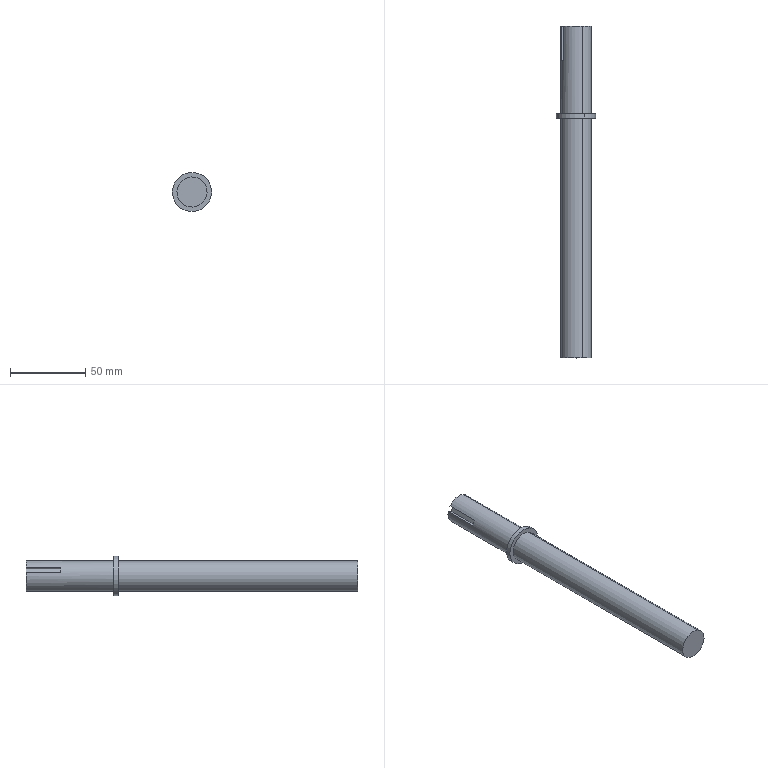Component | SolidWorks | LX-TSJ-07-1 | 1 solid | 18 faces | box 26 x 220 x 26 mm | volume 69227 mm3 | plane 12 | cylinder 6 | commonest cylinder face diameters 20 x4 26 x2
STEP:
#1=COLOUR_RGB('',0.7922,0.8196,0.9333);
#2=FILL_AREA_STYLE_COLOUR('',#1);
#3=FILL_AREA_STYLE('',(#2));
#4=SURFACE_STYLE_FILL_AREA(#3);
#5=SURFACE_SIDE_STYLE('',(#4));
#6=SURFACE_STYLE_USAGE(.BOTH.,#5);
#7=PRESENTATION_STYLE_ASSIGNMENT((#6));
#8=CARTESIAN_POINT('',(-12.95,-27.531,-15.901));
#9=VERTEX_POINT('',#8);
#10=CARTESIAN_POINT('',(-13.272,-27.531,-16.62));
#11=VERTEX_POINT('',#10);
#12=CARTESIAN_POINT('',(-13.111,-27.531,-16.26));
#13=DIRECTION('',(-0.,1.,0.));
#14=DIRECTION('',(0.4092,0.,0.9125));
#15=AXIS2_PLACEMENT_3D('',#12,#13,#14);
#16=CIRCLE('',#15,0.3937);
#17=EDGE_CURVE('',#9,#11,#16,.T.);
#18=ORIENTED_EDGE('',*,*,#17,.T.);
#19=CARTESIAN_POINT('',(-13.272,-21.272,-16.62));
#20=VERTEX_POINT('',#19);
#21=CARTESIAN_POINT('',(-13.272,-18.87,-16.62));
#22=DIRECTION('',(-0.,1.,0.));
#23=VECTOR('',#22,39.37);
#24=LINE('',#21,#23);
#25=EDGE_CURVE('',#11,#20,#24,.T.);
#26=ORIENTED_EDGE('',*,*,#25,.T.);
#27=CARTESIAN_POINT('',(-12.95,-21.272,-15.901));
#28=VERTEX_POINT('',#27);
#29=CARTESIAN_POINT('',(-13.111,-21.272,-16.26));
#30=DIRECTION('',(0.,-1.,-0.));
#31=DIRECTION('',(0.4092,0.,0.9125));
#32=AXIS2_PLACEMENT_3D('',#29,#30,#31);
#33=CIRCLE('',#32,0.3937);
#34=EDGE_CURVE('',#20,#28,#33,.T.);
#35=ORIENTED_EDGE('',*,*,#34,.T.);
#36=CARTESIAN_POINT('',(-12.95,-18.87,-15.901));
#37=DIRECTION('',(-0.,1.,0.));
#38=VECTOR('',#37,39.37);
#39=LINE('',#36,#38);
#40=EDGE_CURVE('',#9,#28,#39,.T.);
#41=ORIENTED_EDGE('',*,*,#40,.F.);
#42=EDGE_LOOP('',(#18,#26,#35,#41));
#43=FACE_OUTER_BOUND('',#42,.T.);
#44=CARTESIAN_POINT('',(-13.111,-18.87,-16.26));
#45=DIRECTION('',(-0.,1.,0.));
#46=DIRECTION('',(0.4092,-0.,0.9125));
#47=AXIS2_PLACEMENT_3D('',#44,#45,#46);
#48=CYLINDRICAL_SURFACE('',#47,0.3937);
#49=ADVANCED_FACE('',(#43),#48,.T.);
#50=CARTESIAN_POINT('',(-13.32,-21.272,-16.727));
#51=VERTEX_POINT('',#50);
#52=CARTESIAN_POINT('',(-12.902,-21.272,-15.793));
#53=VERTEX_POINT('',#52);
#54=CARTESIAN_POINT('',(-13.111,-21.272,-16.26));
#55=DIRECTION('',(0.,-1.,-0.));
#56=DIRECTION('',(0.4092,0.,0.9125));
#57=AXIS2_PLACEMENT_3D('',#54,#55,#56);
#58=CIRCLE('',#57,0.5118);
#59=EDGE_CURVE('',#51,#53,#58,.T.);
#60=ORIENTED_EDGE('',*,*,#59,.F.);
#61=CARTESIAN_POINT('',(-13.32,-21.154,-16.727));
#62=VERTEX_POINT('',#61);
#63=CARTESIAN_POINT('',(-13.32,-18.87,-16.727));
#64=DIRECTION('',(-0.,1.,0.));
#65=VECTOR('',#64,39.37);
#66=LINE('',#63,#65);
#67=EDGE_CURVE('',#51,#62,#66,.T.);
#68=ORIENTED_EDGE('',*,*,#67,.T.);
#69=CARTESIAN_POINT('',(-12.902,-21.154,-15.793));
#70=VERTEX_POINT('',#69);
#71=CARTESIAN_POINT('',(-13.111,-21.154,-16.26));
#72=DIRECTION('',(0.,-1.,-0.));
#73=DIRECTION('',(0.4092,0.,0.9125));
#74=AXIS2_PLACEMENT_3D('',#71,#72,#73);
#75=CIRCLE('',#74,0.5118);
#76=EDGE_CURVE('',#62,#70,#75,.T.);
#77=ORIENTED_EDGE('',*,*,#76,.T.);
#78=CARTESIAN_POINT('',(-12.902,-18.87,-15.793));
#79=DIRECTION('',(-0.,1.,0.));
#80=VECTOR('',#79,39.37);
#81=LINE('',#78,#80);
#82=EDGE_CURVE('',#53,#70,#81,.T.);
#83=ORIENTED_EDGE('',*,*,#82,.F.);
#84=EDGE_LOOP('',(#60,#68,#77,#83));
#85=FACE_OUTER_BOUND('',#84,.T.);
#86=CARTESIAN_POINT('',(-13.111,-18.87,-16.26));
#87=DIRECTION('',(-0.,1.,0.));
#88=DIRECTION('',(0.4092,-0.,0.9125));
#89=AXIS2_PLACEMENT_3D('',#86,#87,#88);
#90=CYLINDRICAL_SURFACE('',#89,0.5118);
#91=ADVANCED_FACE('',(#85),#90,.T.);
#92=CARTESIAN_POINT('',(-13.272,-21.154,-16.62));
#93=VERTEX_POINT('',#92);
#94=CARTESIAN_POINT('',(-12.95,-21.154,-15.901));
#95=VERTEX_POINT('',#94);
#96=CARTESIAN_POINT('',(-13.111,-21.154,-16.26));
#97=DIRECTION('',(0.,-1.,-0.));
#98=DIRECTION('',(0.4092,0.,0.9125));
#99=AXIS2_PLACEMENT_3D('',#96,#97,#98);
#100=CIRCLE('',#99,0.3937);
#101=EDGE_CURVE('',#93,#95,#100,.T.);
#102=ORIENTED_EDGE('',*,*,#101,.F.);
#103=CARTESIAN_POINT('',(-13.272,-18.87,-16.62));
#104=VERTEX_POINT('',#103);
#105=CARTESIAN_POINT('',(-13.272,-18.87,-16.62));
#106=DIRECTION('',(-0.,1.,0.));
#107=VECTOR('',#106,39.37);
#108=LINE('',#105,#107);
#109=EDGE_CURVE('',#93,#104,#108,.T.);
#110=ORIENTED_EDGE('',*,*,#109,.T.);
#111=CARTESIAN_POINT('',(-12.791,-18.87,-16.49));
#112=VERTEX_POINT('',#111);
#113=CARTESIAN_POINT('',(-13.111,-18.87,-16.26));
#114=DIRECTION('',(0.,-1.,-0.));
#115=DIRECTION('',(0.4092,-0.,0.9125));
#116=AXIS2_PLACEMENT_3D('',#113,#114,#115);
#117=CIRCLE('',#116,0.3937);
#118=EDGE_CURVE('',#104,#112,#117,.T.);
#119=ORIENTED_EDGE('',*,*,#118,.T.);
#120=CARTESIAN_POINT('',(-12.791,-19.774,-16.49));
#121=VERTEX_POINT('',#120);
#122=CARTESIAN_POINT('',(-12.791,-18.87,-16.49));
#123=DIRECTION('',(0.,-1.,-0.));
#124=VECTOR('',#123,39.37);
#125=LINE('',#122,#124);
#126=EDGE_CURVE('',#112,#121,#125,.T.);
#127=ORIENTED_EDGE('',*,*,#126,.T.);
#128=CARTESIAN_POINT('',(-12.727,-19.774,-16.346));
#129=VERTEX_POINT('',#128);
#130=CARTESIAN_POINT('',(-13.111,-19.774,-16.26));
#131=DIRECTION('',(0.,-1.,-0.));
#132=DIRECTION('',(0.4092,0.,0.9125));
#133=AXIS2_PLACEMENT_3D('',#130,#131,#132);
#134=CIRCLE('',#133,0.3937);
#135=EDGE_CURVE('',#121,#129,#134,.T.);
#136=ORIENTED_EDGE('',*,*,#135,.T.);
#137=CARTESIAN_POINT('',(-12.727,-18.87,-16.346));
#138=VERTEX_POINT('',#137);
#139=CARTESIAN_POINT('',(-12.727,-18.87,-16.346));
#140=DIRECTION('',(-0.,1.,0.));
#141=VECTOR('',#140,39.37);
#142=LINE('',#139,#141);
#143=EDGE_CURVE('',#129,#138,#142,.T.);
#144=ORIENTED_EDGE('',*,*,#143,.T.);
#145=CARTESIAN_POINT('',(-12.95,-18.87,-15.901));
#146=VERTEX_POINT('',#145);
#147=CARTESIAN_POINT('',(-13.111,-18.87,-16.26));
#148=DIRECTION('',(0.,-1.,-0.));
#149=DIRECTION('',(0.4092,-0.,0.9125));
#150=AXIS2_PLACEMENT_3D('',#147,#148,#149);
#151=CIRCLE('',#150,0.3937);
#152=EDGE_CURVE('',#138,#146,#151,.T.);
#153=ORIENTED_EDGE('',*,*,#152,.T.);
#154=CARTESIAN_POINT('',(-12.95,-18.87,-15.901));
#155=DIRECTION('',(-0.,1.,0.));
#156=VECTOR('',#155,39.37);
#157=LINE('',#154,#156);
#158=EDGE_CURVE('',#95,#146,#157,.T.);
#159=ORIENTED_EDGE('',*,*,#158,.F.);
#160=EDGE_LOOP('',(#102,#110,#119,#127,#136,#144,#153,#159));
#161=FACE_OUTER_BOUND('',#160,.T.);
#162=CARTESIAN_POINT('',(-13.111,-18.87,-16.26));
#163=DIRECTION('',(-0.,1.,0.));
#164=DIRECTION('',(0.4092,-0.,0.9125));
#165=AXIS2_PLACEMENT_3D('',#162,#163,#164);
#166=CYLINDRICAL_SURFACE('',#165,0.3937);
#167=ADVANCED_FACE('',(#161),#166,.T.);
#168=ORIENTED_EDGE('',*,*,#25,.F.);
#169=CARTESIAN_POINT('',(-13.111,-27.531,-16.26));
#170=DIRECTION('',(-0.,1.,0.));
#171=DIRECTION('',(0.4092,0.,0.9125));
#172=AXIS2_PLACEMENT_3D('',#169,#170,#171);
#173=CIRCLE('',#172,0.3937);
#174=EDGE_CURVE('',#11,#9,#173,.T.);
#175=ORIENTED_EDGE('',*,*,#174,.T.);
#176=ORIENTED_EDGE('',*,*,#40,.T.);
#177=CARTESIAN_POINT('',(-13.111,-21.272,-16.26));
#178=DIRECTION('',(0.,-1.,-0.));
#179=DIRECTION('',(0.4092,0.,0.9125));
#180=AXIS2_PLACEMENT_3D('',#177,#178,#179);
#181=CIRCLE('',#180,0.3937);
#182=EDGE_CURVE('',#28,#20,#181,.T.);
#183=ORIENTED_EDGE('',*,*,#182,.T.);
#184=EDGE_LOOP('',(#168,#175,#176,#183));
#185=FACE_OUTER_BOUND('',#184,.T.);
#186=CARTESIAN_POINT('',(-13.111,-18.87,-16.26));
#187=DIRECTION('',(-0.,1.,0.));
#188=DIRECTION('',(0.4092,-0.,0.9125));
#189=AXIS2_PLACEMENT_3D('',#186,#187,#188);
#190=CYLINDRICAL_SURFACE('',#189,0.3937);
#191=ADVANCED_FACE('',(#185),#190,.T.);
#192=CARTESIAN_POINT('',(-13.111,-21.272,-16.26));
#193=DIRECTION('',(0.,-1.,-0.));
#194=DIRECTION('',(0.4092,0.,0.9125));
#195=AXIS2_PLACEMENT_3D('',#192,#193,#194);
#196=CIRCLE('',#195,0.5118);
#197=EDGE_CURVE('',#53,#51,#196,.T.);
#198=ORIENTED_EDGE('',*,*,#197,.T.);
#199=ORIENTED_EDGE('',*,*,#59,.T.);
#200=EDGE_LOOP('',(#198,#199));
#201=FACE_OUTER_BOUND('',#200,.T.);
#202=ORIENTED_EDGE('',*,*,#182,.F.);
#203=ORIENTED_EDGE('',*,*,#34,.F.);
#204=EDGE_LOOP('',(#202,#203));
#205=FACE_BOUND('',#204,.T.);
#206=CARTESIAN_POINT('',(-13.954,-21.272,-15.882));
#207=DIRECTION('',(0.,-1.,-0.));
#208=DIRECTION('',(-0.4092,0.,-0.9125));
#209=AXIS2_PLACEMENT_3D('',#206,#207,#208);
#210=PLANE('',#209);
#211=ADVANCED_FACE('',(#201,#205),#210,.T.);
#212=ORIENTED_EDGE('',*,*,#17,.F.);
#213=ORIENTED_EDGE('',*,*,#174,.F.);
#214=EDGE_LOOP('',(#212,#213));
#215=FACE_OUTER_BOUND('',#214,.T.);
#216=CARTESIAN_POINT('',(-13.954,-27.531,-15.882));
#217=DIRECTION('',(0.,-1.,-0.));
#218=DIRECTION('',(-0.4092,0.,-0.9125));
#219=AXIS2_PLACEMENT_3D('',#216,#217,#218);
#220=PLANE('',#219);
#221=ADVANCED_FACE('',(#215),#220,.T.);
#222=ORIENTED_EDGE('',*,*,#67,.F.);
#223=ORIENTED_EDGE('',*,*,#197,.F.);
#224=ORIENTED_EDGE('',*,*,#82,.T.);
#225=CARTESIAN_POINT('',(-13.111,-21.154,-16.26));
#226=DIRECTION('',(0.,-1.,-0.));
#227=DIRECTION('',(0.4092,0.,0.9125));
#228=AXIS2_PLACEMENT_3D('',#225,#226,#227);
#229=CIRCLE('',#228,0.5118);
#230=EDGE_CURVE('',#70,#62,#229,.T.);
#231=ORIENTED_EDGE('',*,*,#230,.T.);
#232=EDGE_LOOP('',(#222,#223,#224,#231));
#233=FACE_OUTER_BOUND('',#232,.T.);
#234=CARTESIAN_POINT('',(-13.111,-18.87,-16.26));
#235=DIRECTION('',(-0.,1.,0.));
#236=DIRECTION('',(0.4092,-0.,0.9125));
#237=AXIS2_PLACEMENT_3D('',#234,#235,#236);
#238=CYLINDRICAL_SURFACE('',#237,0.5118);
#239=ADVANCED_FACE('',(#233),#238,.T.);
#240=CARTESIAN_POINT('',(-13.111,-21.154,-16.26));
#241=DIRECTION('',(0.,-1.,-0.));
#242=DIRECTION('',(0.4092,0.,0.9125));
#243=AXIS2_PLACEMENT_3D('',#240,#241,#242);
#244=CIRCLE('',#243,0.3937);
#245=EDGE_CURVE('',#95,#93,#244,.T.);
#246=ORIENTED_EDGE('',*,*,#245,.T.);
#247=ORIENTED_EDGE('',*,*,#101,.T.);
#248=EDGE_LOOP('',(#246,#247));
#249=FACE_BOUND('',#248,.T.);
#250=ORIENTED_EDGE('',*,*,#230,.F.);
#251=ORIENTED_EDGE('',*,*,#76,.F.);
#252=EDGE_LOOP('',(#250,#251));
#253=FACE_OUTER_BOUND('',#252,.T.);
#254=CARTESIAN_POINT('',(-13.954,-21.154,-15.882));
#255=DIRECTION('',(-0.,1.,0.));
#256=DIRECTION('',(0.4092,-0.,0.9125));
#257=AXIS2_PLACEMENT_3D('',#254,#255,#256);
#258=PLANE('',#257);
#259=ADVANCED_FACE('',(#249,#253),#258,.T.);
#260=ORIENTED_EDGE('',*,*,#109,.F.);
#261=ORIENTED_EDGE('',*,*,#245,.F.);
#262=ORIENTED_EDGE('',*,*,#158,.T.);
#263=CARTESIAN_POINT('',(-13.431,-18.87,-16.031));
#264=VERTEX_POINT('',#263);
#265=CARTESIAN_POINT('',(-13.111,-18.87,-16.26));
#266=DIRECTION('',(0.,-1.,-0.));
#267=DIRECTION('',(0.4092,-0.,0.9125));
#268=AXIS2_PLACEMENT_3D('',#265,#266,#267);
#269=CIRCLE('',#268,0.3937);
#270=EDGE_CURVE('',#146,#264,#269,.T.);
#271=ORIENTED_EDGE('',*,*,#270,.T.);
#272=CARTESIAN_POINT('',(-13.431,-19.774,-16.031));
#273=VERTEX_POINT('',#272);
#274=CARTESIAN_POINT('',(-13.431,-18.87,-16.031));
#275=DIRECTION('',(0.,-1.,-0.));
#276=VECTOR('',#275,39.37);
#277=LINE('',#274,#276);
#278=EDGE_CURVE('',#264,#273,#277,.T.);
#279=ORIENTED_EDGE('',*,*,#278,.T.);
#280=CARTESIAN_POINT('',(-13.495,-19.774,-16.174));
#281=VERTEX_POINT('',#280);
#282=CARTESIAN_POINT('',(-13.111,-19.774,-16.26));
#283=DIRECTION('',(0.,-1.,-0.));
#284=DIRECTION('',(0.4092,0.,0.9125));
#285=AXIS2_PLACEMENT_3D('',#282,#283,#284);
#286=CIRCLE('',#285,0.3937);
#287=EDGE_CURVE('',#273,#281,#286,.T.);
#288=ORIENTED_EDGE('',*,*,#287,.T.);
#289=CARTESIAN_POINT('',(-13.495,-18.87,-16.174));
#290=VERTEX_POINT('',#289);
#291=CARTESIAN_POINT('',(-13.495,-18.87,-16.174));
#292=DIRECTION('',(-0.,1.,0.));
#293=VECTOR('',#292,39.37);
#294=LINE('',#291,#293);
#295=EDGE_CURVE('',#281,#290,#294,.T.);
#296=ORIENTED_EDGE('',*,*,#295,.T.);
#297=CARTESIAN_POINT('',(-13.111,-18.87,-16.26));
#298=DIRECTION('',(0.,-1.,-0.));
#299=DIRECTION('',(0.4092,-0.,0.9125));
#300=AXIS2_PLACEMENT_3D('',#297,#298,#299);
#301=CIRCLE('',#300,0.3937);
#302=EDGE_CURVE('',#290,#104,#301,.T.);
#303=ORIENTED_EDGE('',*,*,#302,.T.);
#304=EDGE_LOOP('',(#260,#261,#262,#271,#279,#288,#296,#303));
#305=FACE_OUTER_BOUND('',#304,.T.);
#306=CARTESIAN_POINT('',(-13.111,-18.87,-16.26));
#307=DIRECTION('',(-0.,1.,0.));
#308=DIRECTION('',(0.4092,-0.,0.9125));
#309=AXIS2_PLACEMENT_3D('',#306,#307,#308);
#310=CYLINDRICAL_SURFACE('',#309,0.3937);
#311=ADVANCED_FACE('',(#305),#310,.T.);
#312=CARTESIAN_POINT('',(-12.827,-18.87,-16.301));
#313=VERTEX_POINT('',#312);
#314=CARTESIAN_POINT('',(-12.892,-18.87,-16.445));
#315=VERTEX_POINT('',#314);
#316=CARTESIAN_POINT('',(-12.859,-18.87,-16.373));
#317=DIRECTION('',(-0.4092,0.,-0.9125));
#318=VECTOR('',#317,39.37);
#319=LINE('',#316,#318);
#320=EDGE_CURVE('',#313,#315,#319,.T.);
#321=ORIENTED_EDGE('',*,*,#320,.T.);
#322=CARTESIAN_POINT('',(-13.986,-18.87,-15.954));
#323=DIRECTION('',(0.9125,0.,-0.4092));
#324=VECTOR('',#323,39.37);
#325=LINE('',#322,#324);
#326=EDGE_CURVE('',#315,#112,#325,.T.);
#327=ORIENTED_EDGE('',*,*,#326,.T.);
#328=ORIENTED_EDGE('',*,*,#118,.F.);
#329=ORIENTED_EDGE('',*,*,#302,.F.);
#330=CARTESIAN_POINT('',(-13.395,-18.87,-16.22));
#331=VERTEX_POINT('',#330);
#332=CARTESIAN_POINT('',(-13.986,-18.87,-15.954));
#333=DIRECTION('',(0.9125,0.,-0.4092));
#334=VECTOR('',#333,39.37);
#335=LINE('',#332,#334);
#336=EDGE_CURVE('',#290,#331,#335,.T.);
#337=ORIENTED_EDGE('',*,*,#336,.T.);
#338=CARTESIAN_POINT('',(-13.33,-18.87,-16.076));
#339=VERTEX_POINT('',#338);
#340=CARTESIAN_POINT('',(-13.362,-18.87,-16.148));
#341=DIRECTION('',(0.4092,-0.,0.9125));
#342=VECTOR('',#341,39.37);
#343=LINE('',#340,#342);
#344=EDGE_CURVE('',#331,#339,#343,.T.);
#345=ORIENTED_EDGE('',*,*,#344,.T.);
#346=CARTESIAN_POINT('',(-13.922,-18.87,-15.81));
#347=DIRECTION('',(-0.9125,-0.,0.4092));
#348=VECTOR('',#347,39.37);
#349=LINE('',#346,#348);
#350=EDGE_CURVE('',#339,#264,#349,.T.);
#351=ORIENTED_EDGE('',*,*,#350,.T.);
#352=ORIENTED_EDGE('',*,*,#270,.F.);
#353=ORIENTED_EDGE('',*,*,#152,.F.);
#354=CARTESIAN_POINT('',(-13.922,-18.87,-15.81));
#355=DIRECTION('',(-0.9125,-0.,0.4092));
#356=VECTOR('',#355,39.37);
#357=LINE('',#354,#356);
#358=EDGE_CURVE('',#138,#313,#357,.T.);
#359=ORIENTED_EDGE('',*,*,#358,.T.);
#360=EDGE_LOOP('',(#321,#327,#328,#329,#337,#345,#351,#352,#353,#359));
#361=FACE_OUTER_BOUND('',#360,.T.);
#362=CARTESIAN_POINT('',(-13.954,-18.87,-15.882));
#363=DIRECTION('',(-0.,1.,0.));
#364=DIRECTION('',(0.4092,-0.,0.9125));
#365=AXIS2_PLACEMENT_3D('',#362,#363,#364);
#366=PLANE('',#365);
#367=ADVANCED_FACE('',(#361),#366,.T.);
#368=CARTESIAN_POINT('',(-13.395,-19.774,-16.22));
#369=VERTEX_POINT('',#368);
#370=CARTESIAN_POINT('',(-13.986,-19.774,-15.954));
#371=DIRECTION('',(0.9125,0.,-0.4092));
#372=VECTOR('',#371,39.37);
#373=LINE('',#370,#372);
#374=EDGE_CURVE('',#281,#369,#373,.T.);
#375=ORIENTED_EDGE('',*,*,#374,.T.);
#376=CARTESIAN_POINT('',(-13.395,-19.774,-16.22));
#377=DIRECTION('',(-0.,1.,0.));
#378=VECTOR('',#377,39.37);
#379=LINE('',#376,#378);
#380=EDGE_CURVE('',#369,#331,#379,.T.);
#381=ORIENTED_EDGE('',*,*,#380,.T.);
#382=ORIENTED_EDGE('',*,*,#336,.F.);
#383=ORIENTED_EDGE('',*,*,#295,.F.);
#384=EDGE_LOOP('',(#375,#381,#382,#383));
#385=FACE_OUTER_BOUND('',#384,.T.);
#386=CARTESIAN_POINT('',(-13.986,-19.774,-15.954));
#387=DIRECTION('',(0.4092,-0.,0.9125));
#388=DIRECTION('',(0.,-1.,-0.));
#389=AXIS2_PLACEMENT_3D('',#386,#387,#388);
#390=PLANE('',#389);
#391=ADVANCED_FACE('',(#385),#390,.T.);
#392=CARTESIAN_POINT('',(-13.33,-19.774,-16.076));
#393=VERTEX_POINT('',#392);
#394=CARTESIAN_POINT('',(-13.362,-19.774,-16.148));
#395=DIRECTION('',(-0.4092,0.,-0.9125));
#396=VECTOR('',#395,39.37);
#397=LINE('',#394,#396);
#398=EDGE_CURVE('',#393,#369,#397,.T.);
#399=ORIENTED_EDGE('',*,*,#398,.T.);
#400=ORIENTED_EDGE('',*,*,#374,.F.);
#401=ORIENTED_EDGE('',*,*,#287,.F.);
#402=CARTESIAN_POINT('',(-13.922,-19.774,-15.81));
#403=DIRECTION('',(0.9125,0.,-0.4092));
#404=VECTOR('',#403,39.37);
#405=LINE('',#402,#404);
#406=EDGE_CURVE('',#273,#393,#405,.T.);
#407=ORIENTED_EDGE('',*,*,#406,.T.);
#408=EDGE_LOOP('',(#399,#400,#401,#407));
#409=FACE_OUTER_BOUND('',#408,.T.);
#410=CARTESIAN_POINT('',(-13.954,-19.774,-15.882));
#411=DIRECTION('',(-0.,1.,0.));
#412=DIRECTION('',(0.4092,-0.,0.9125));
#413=AXIS2_PLACEMENT_3D('',#410,#411,#412);
#414=PLANE('',#413);
#415=ADVANCED_FACE('',(#409),#414,.T.);
#416=CARTESIAN_POINT('',(-13.33,-19.774,-16.076));
#417=DIRECTION('',(-0.,1.,0.));
#418=VECTOR('',#417,39.37);
#419=LINE('',#416,#418);
#420=EDGE_CURVE('',#393,#339,#419,.T.);
#421=ORIENTED_EDGE('',*,*,#420,.F.);
#422=ORIENTED_EDGE('',*,*,#406,.F.);
#423=ORIENTED_EDGE('',*,*,#278,.F.);
#424=ORIENTED_EDGE('',*,*,#350,.F.);
#425=EDGE_LOOP('',(#421,#422,#423,#424));
#426=FACE_OUTER_BOUND('',#425,.T.);
#427=CARTESIAN_POINT('',(-13.922,-19.774,-15.81));
#428=DIRECTION('',(0.4092,-0.,0.9125));
#429=DIRECTION('',(0.,-1.,-0.));
#430=AXIS2_PLACEMENT_3D('',#427,#428,#429);
#431=PLANE('',#430);
#432=ADVANCED_FACE('',(#426),#431,.F.);
#433=ORIENTED_EDGE('',*,*,#143,.F.);
#434=CARTESIAN_POINT('',(-12.827,-19.774,-16.301));
#435=VERTEX_POINT('',#434);
#436=CARTESIAN_POINT('',(-13.922,-19.774,-15.81));
#437=DIRECTION('',(0.9125,0.,-0.4092));
#438=VECTOR('',#437,39.37);
#439=LINE('',#436,#438);
#440=EDGE_CURVE('',#435,#129,#439,.T.);
#441=ORIENTED_EDGE('',*,*,#440,.F.);
#442=CARTESIAN_POINT('',(-12.827,-19.774,-16.301));
#443=DIRECTION('',(0.,-1.,-0.));
#444=VECTOR('',#443,39.37);
#445=LINE('',#442,#444);
#446=EDGE_CURVE('',#313,#435,#445,.T.);
#447=ORIENTED_EDGE('',*,*,#446,.F.);
#448=ORIENTED_EDGE('',*,*,#358,.F.);
#449=EDGE_LOOP('',(#433,#441,#447,#448));
#450=FACE_OUTER_BOUND('',#449,.T.);
#451=CARTESIAN_POINT('',(-13.922,-19.774,-15.81));
#452=DIRECTION('',(0.4092,-0.,0.9125));
#453=DIRECTION('',(0.,-1.,-0.));
#454=AXIS2_PLACEMENT_3D('',#451,#452,#453);
#455=PLANE('',#454);
#456=ADVANCED_FACE('',(#450),#455,.F.);
#457=ORIENTED_EDGE('',*,*,#440,.T.);
#458=ORIENTED_EDGE('',*,*,#135,.F.);
#459=CARTESIAN_POINT('',(-12.892,-19.774,-16.445));
#460=VERTEX_POINT('',#459);
#461=CARTESIAN_POINT('',(-13.986,-19.774,-15.954));
#462=DIRECTION('',(-0.9125,-0.,0.4092));
#463=VECTOR('',#462,39.37);
#464=LINE('',#461,#463);
#465=EDGE_CURVE('',#121,#460,#464,.T.);
#466=ORIENTED_EDGE('',*,*,#465,.T.);
#467=CARTESIAN_POINT('',(-12.859,-19.774,-16.373));
#468=DIRECTION('',(0.4092,-0.,0.9125));
#469=VECTOR('',#468,39.37);
#470=LINE('',#467,#469);
#471=EDGE_CURVE('',#460,#435,#470,.T.);
#472=ORIENTED_EDGE('',*,*,#471,.T.);
#473=EDGE_LOOP('',(#457,#458,#466,#472));
#474=FACE_OUTER_BOUND('',#473,.T.);
#475=CARTESIAN_POINT('',(-13.954,-19.774,-15.882));
#476=DIRECTION('',(-0.,1.,0.));
#477=DIRECTION('',(0.4092,-0.,0.9125));
#478=AXIS2_PLACEMENT_3D('',#475,#476,#477);
#479=PLANE('',#478);
#480=ADVANCED_FACE('',(#474),#479,.T.);
#481=ORIENTED_EDGE('',*,*,#465,.F.);
#482=ORIENTED_EDGE('',*,*,#126,.F.);
#483=ORIENTED_EDGE('',*,*,#326,.F.);
#484=CARTESIAN_POINT('',(-12.892,-19.774,-16.445));
#485=DIRECTION('',(0.,-1.,-0.));
#486=VECTOR('',#485,39.37);
#487=LINE('',#484,#486);
#488=EDGE_CURVE('',#315,#460,#487,.T.);
#489=ORIENTED_EDGE('',*,*,#488,.T.);
#490=EDGE_LOOP('',(#481,#482,#483,#489));
#491=FACE_OUTER_BOUND('',#490,.T.);
#492=CARTESIAN_POINT('',(-13.986,-19.774,-15.954));
#493=DIRECTION('',(0.4092,-0.,0.9125));
#494=DIRECTION('',(0.,-1.,-0.));
#495=AXIS2_PLACEMENT_3D('',#492,#493,#494);
#496=PLANE('',#495);
#497=ADVANCED_FACE('',(#491),#496,.T.);
#498=ORIENTED_EDGE('',*,*,#471,.F.);
#499=ORIENTED_EDGE('',*,*,#488,.F.);
#500=ORIENTED_EDGE('',*,*,#320,.F.);
#501=ORIENTED_EDGE('',*,*,#446,.T.);
#502=EDGE_LOOP('',(#498,#499,#500,#501));
#503=FACE_OUTER_BOUND('',#502,.T.);
#504=CARTESIAN_POINT('',(-12.859,-19.774,-16.373));
#505=DIRECTION('',(0.9125,0.,-0.4092));
#506=DIRECTION('',(0.4092,-0.,0.9125));
#507=AXIS2_PLACEMENT_3D('',#504,#505,#506);
#508=PLANE('',#507);
#509=ADVANCED_FACE('',(#503),#508,.T.);
#510=ORIENTED_EDGE('',*,*,#398,.F.);
#511=ORIENTED_EDGE('',*,*,#420,.T.);
#512=ORIENTED_EDGE('',*,*,#344,.F.);
#513=ORIENTED_EDGE('',*,*,#380,.F.);
#514=EDGE_LOOP('',(#510,#511,#512,#513));
#515=FACE_OUTER_BOUND('',#514,.T.);
#516=CARTESIAN_POINT('',(-13.362,-19.774,-16.148));
#517=DIRECTION('',(-0.9125,-0.,0.4092));
#518=DIRECTION('',(-0.4092,0.,-0.9125));
#519=AXIS2_PLACEMENT_3D('',#516,#517,#518);
#520=PLANE('',#519);
#521=ADVANCED_FACE('',(#515),#520,.T.);
#522=CLOSED_SHELL('',(#49,#91,#167,#191,#211,#221,#239,#259,#311,#367,#391,#415,#432,#456,#480,#497,#509,#521));
#523=MANIFOLD_SOLID_BREP('',#522);
#524=STYLED_ITEM('',(#7),#523);
#525=PRESENTATION_LAYER_ASSIGNMENT('','',(#524));
#526=CARTESIAN_POINT('',(0.,0.,0.));
#527=DIRECTION('',(0.,0.,1.));
#528=DIRECTION('',(1.,0.,0.));
#529=AXIS2_PLACEMENT_3D('',#526,#527,#528);
#530=(LENGTH_UNIT()NAMED_UNIT(*)SI_UNIT($,.METRE.));
#531=LENGTH_MEASURE_WITH_UNIT(LENGTH_MEASURE(0.0254),#530);
#532=DIMENSIONAL_EXPONENTS(1.,0.,0.,0.,0.,0.,0.);
#533=(CONVERSION_BASED_UNIT('',#531)LENGTH_UNIT()NAMED_UNIT(#532));
#534=UNCERTAINTY_MEASURE_WITH_UNIT(LENGTH_MEASURE(0.00001),#533,'','');
#535=(NAMED_UNIT(*)PLANE_ANGLE_UNIT()SI_UNIT($,.RADIAN.));
#536=(NAMED_UNIT(*)SI_UNIT($,.STERADIAN.)SOLID_ANGLE_UNIT());
#537=(GEOMETRIC_REPRESENTATION_CONTEXT(3)GLOBAL_UNCERTAINTY_ASSIGNED_CONTEXT((#534))GLOBAL_UNIT_ASSIGNED_CONTEXT((#533,#535,#536))REPRESENTATION_CONTEXT('',''));
#538=ADVANCED_BREP_SHAPE_REPRESENTATION('',(#523,#529),#537);
#539=(LENGTH_UNIT()NAMED_UNIT(*)SI_UNIT($,.METRE.));
#540=LENGTH_MEASURE_WITH_UNIT(LENGTH_MEASURE(0.0254),#539);
#541=DIMENSIONAL_EXPONENTS(1.,0.,0.,0.,0.,0.,0.);
#542=(CONVERSION_BASED_UNIT('',#540)LENGTH_UNIT()NAMED_UNIT(#541));
#543=UNCERTAINTY_MEASURE_WITH_UNIT(LENGTH_MEASURE(0.00001),#542,'','');
#544=(NAMED_UNIT(*)PLANE_ANGLE_UNIT()SI_UNIT($,.RADIAN.));
#545=(NAMED_UNIT(*)SI_UNIT($,.STERADIAN.)SOLID_ANGLE_UNIT());
#546=(GEOMETRIC_REPRESENTATION_CONTEXT(3)GLOBAL_UNCERTAINTY_ASSIGNED_CONTEXT((#543))GLOBAL_UNIT_ASSIGNED_CONTEXT((#542,#544,#545))REPRESENTATION_CONTEXT('',''));
#547=MECHANICAL_DESIGN_GEOMETRIC_PRESENTATION_REPRESENTATION('',(#524),#546);